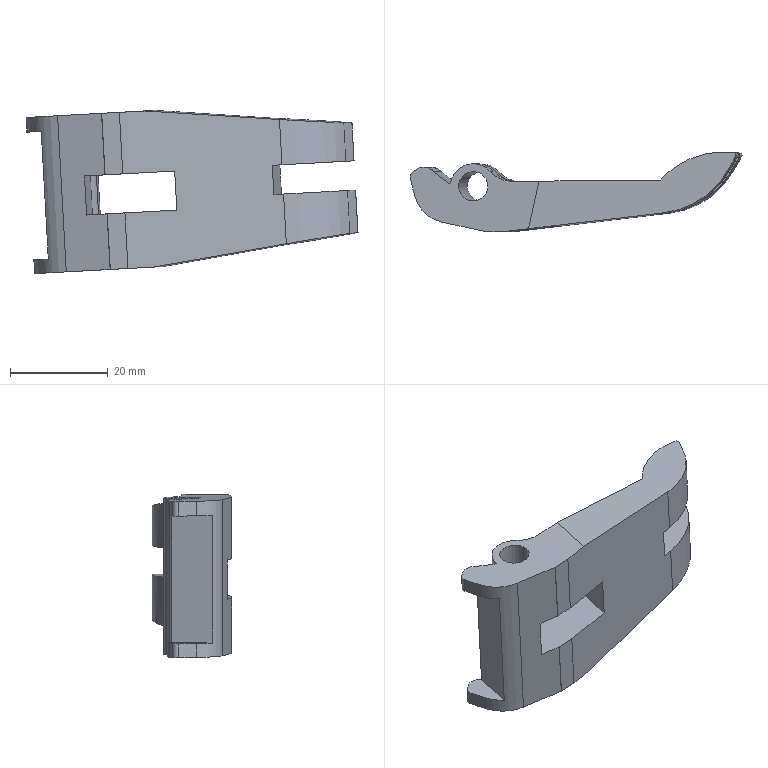Component | NX | LEVER_3 | 1 solid | 44 faces | volume 13530 mm3 | plane 26 | cylinder 18 | commonest cylinder face diameters 4.749 x2 1.306 x2 34.787 x2 16 x2 12 x2 2.306 x2 33.697 x1 9.208 x1